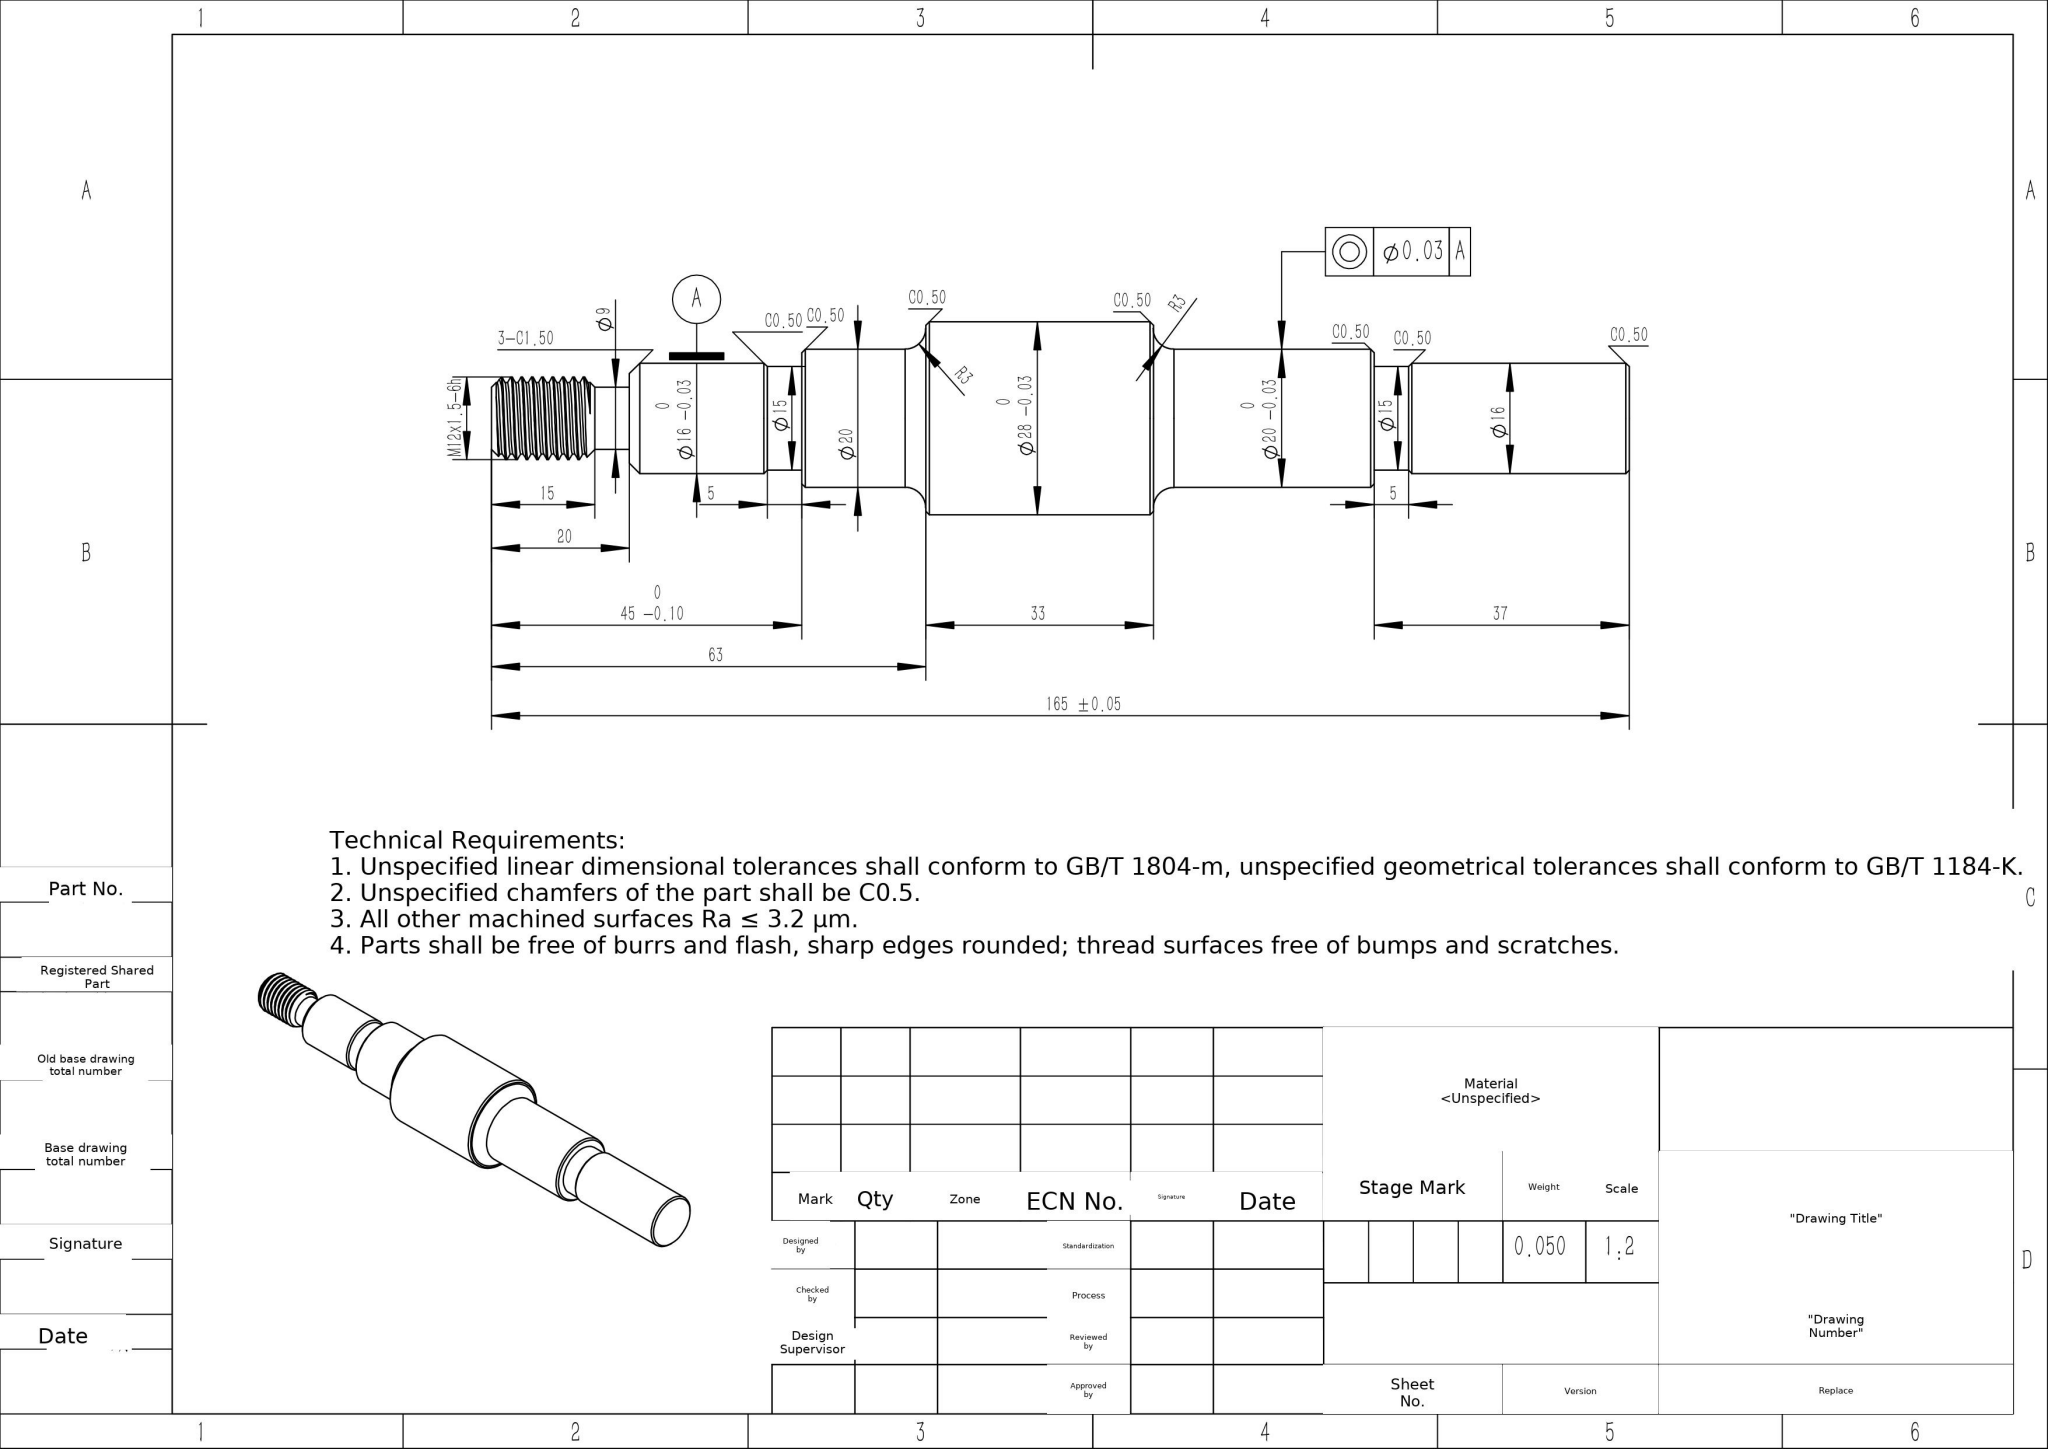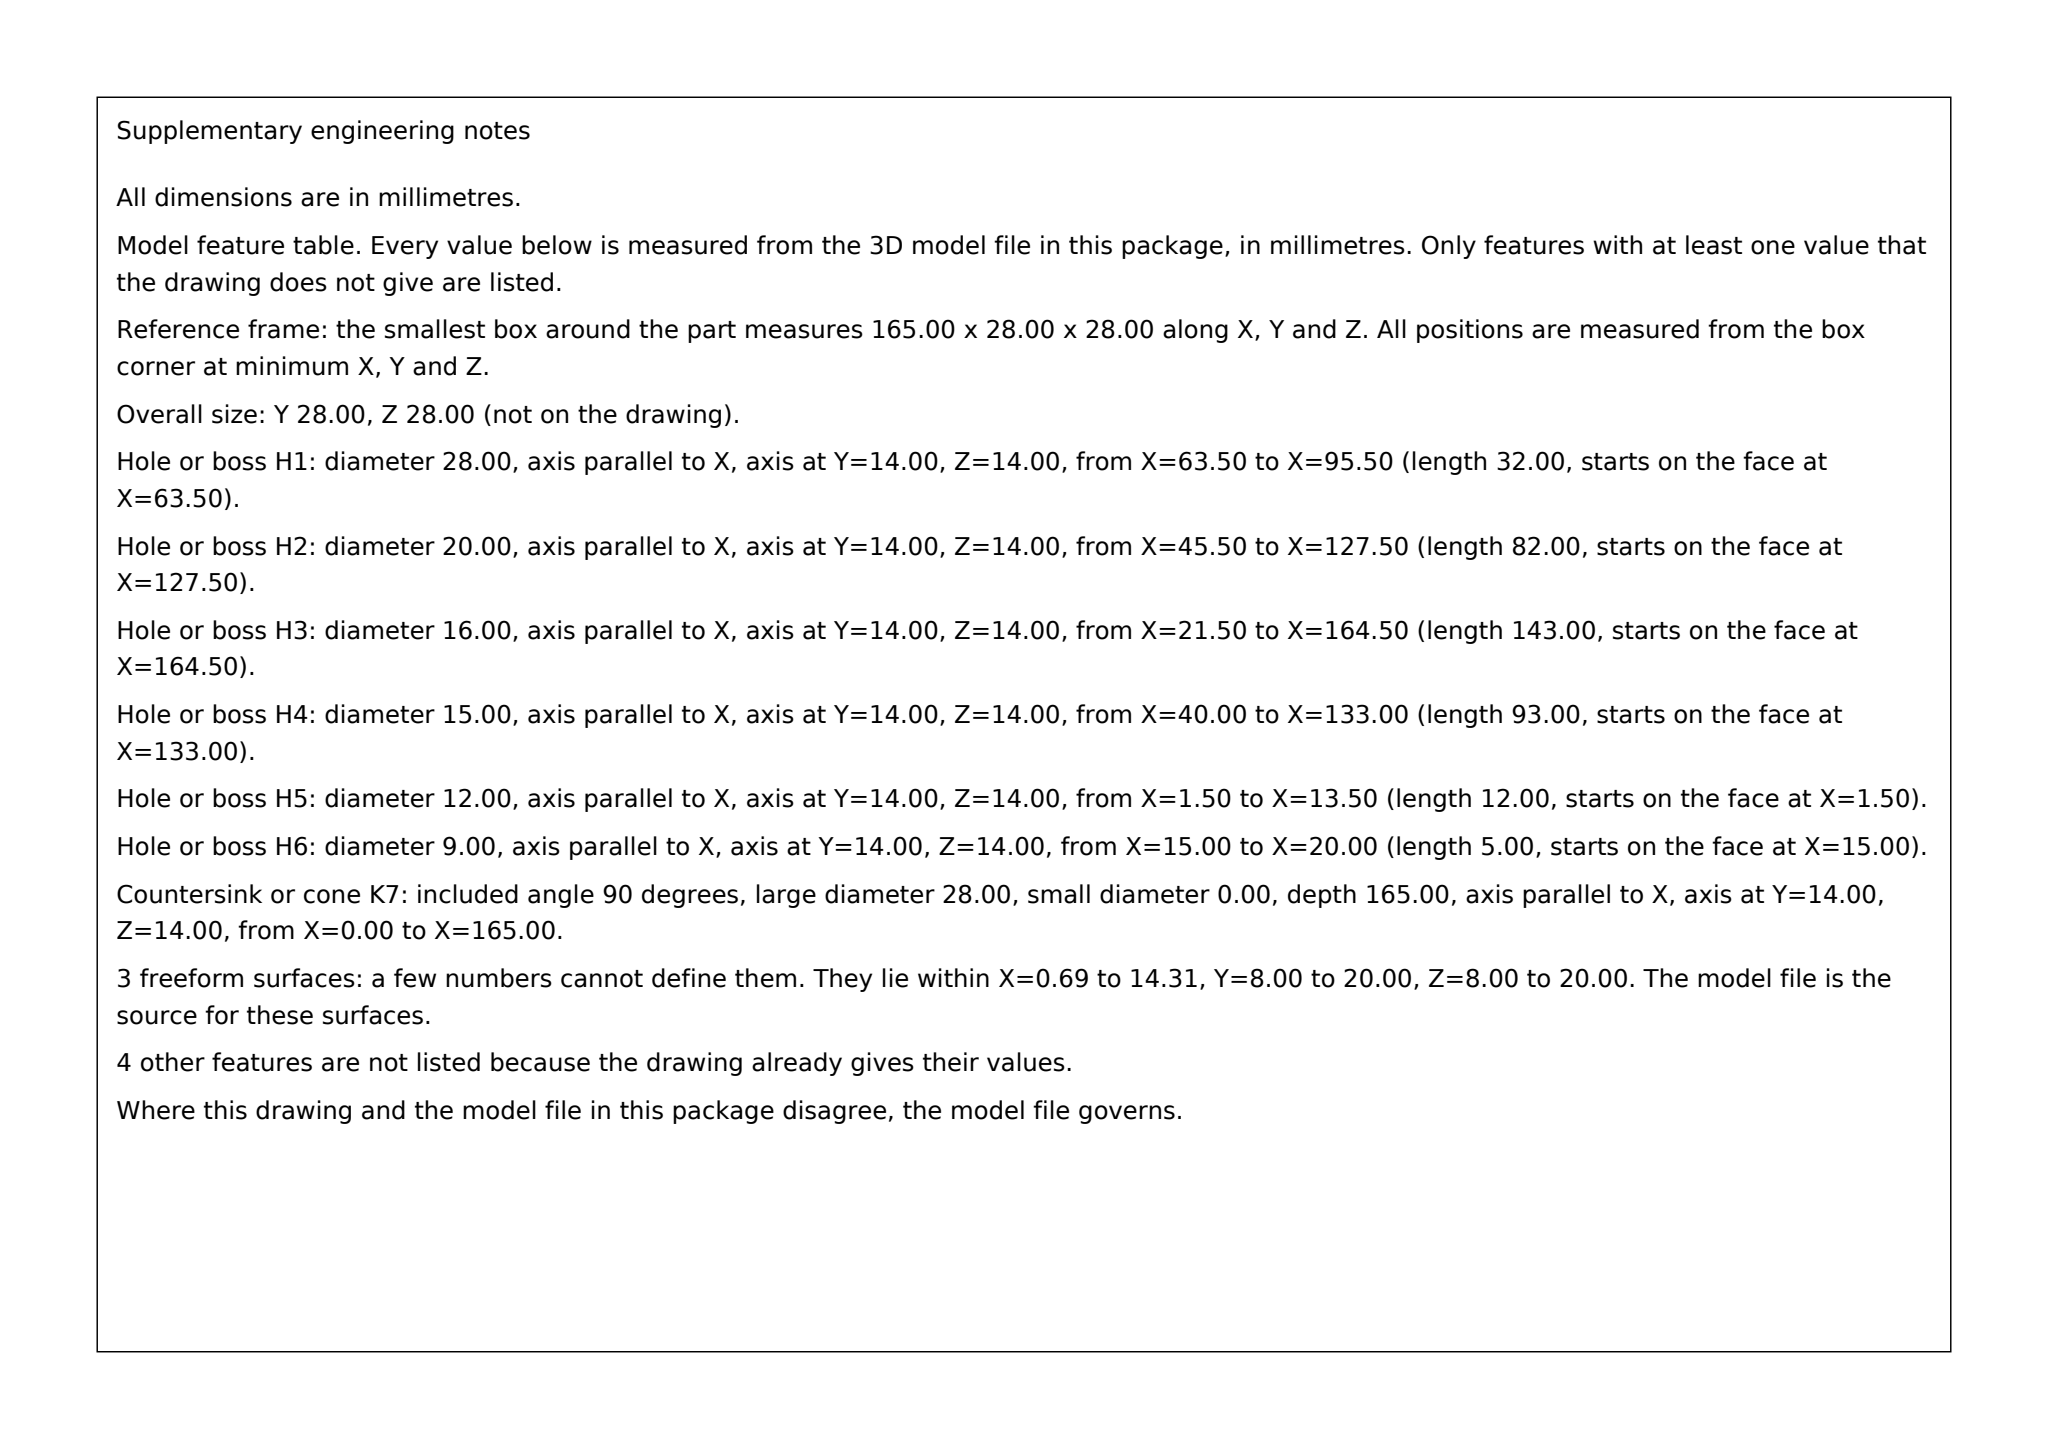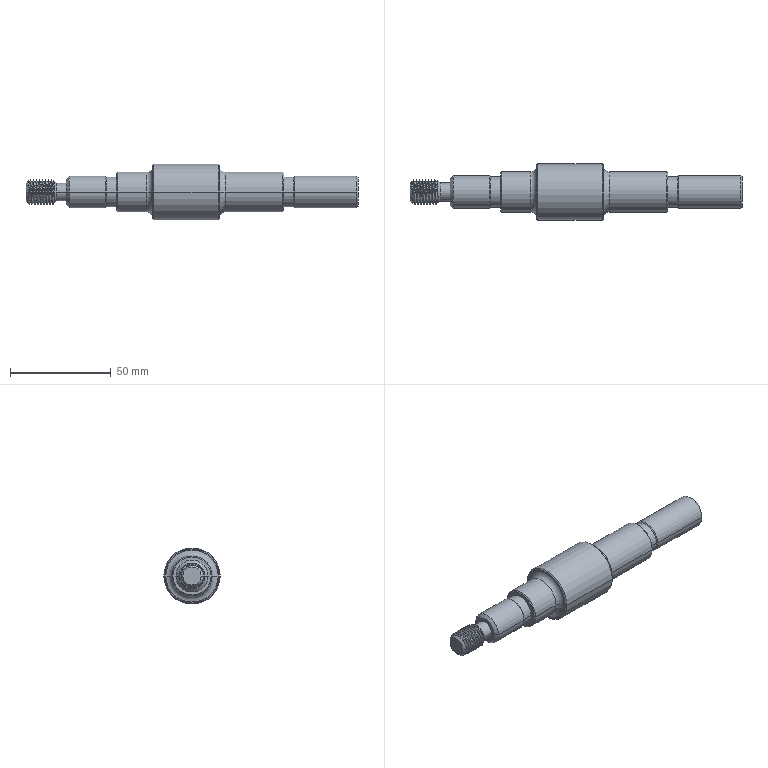Part | SolidWorks | mm | 1 solid | 67 faces | box 165 x 28 x 28 mm | volume 50135 mm3 | cylinder 33 | cone 20 | plane 7 | torus 4 | spline 3 | commonest cylinder face diameters 12 x17 16 x4 15 x4 20 x4 28 x2 9 x2